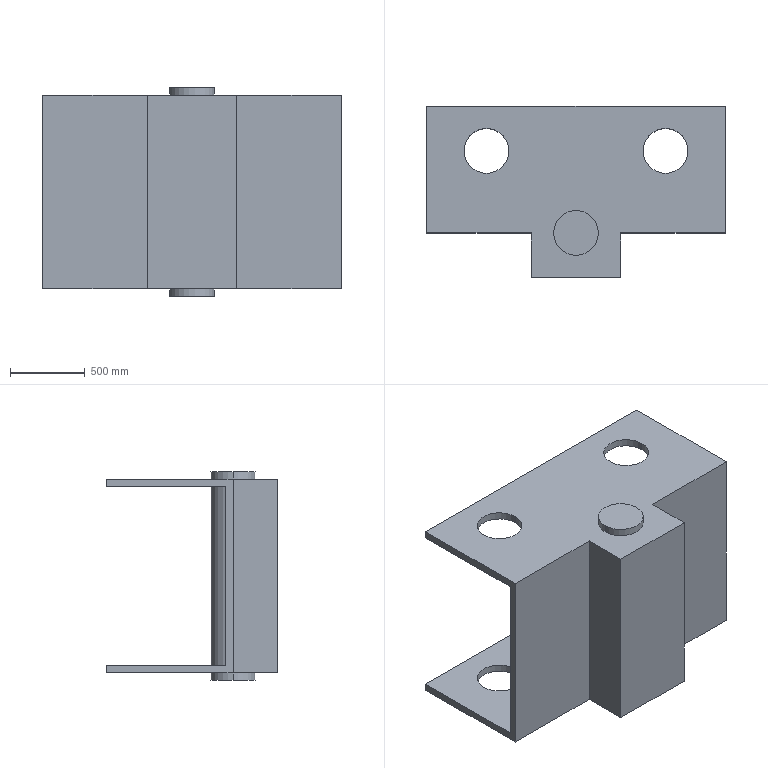Component | SolidWorks | RunningMechanism-4_Part12-2 | 1 solid | 34 faces | box 2000 x 1150 x 1400 mm | volume 421754418 mm3 | plane 20 | cylinder 14 | commonest cylinder face diameters 300 x14
build123d program:
from build123d import *

# Parameters (mm, degrees)
BOSS_EXTRUDE1_DEPTH = 650
SHELL1_T            = -50
SKETCH2_R           = 150
CUT_EXTRUDE1_DEPTH  = 1300
BOSS_EXTRUDE2_START = 50
SKETCH3_R           = 150
BOSS_EXTRUDE2_DEPTH = 1400


with BuildPart() as part:
    # Sketch1 → Boss-Extrude1 (new, symmetric)
    with BuildSketch(Plane(origin=(0, 0, 0), x_dir=(0, 0, -1), z_dir=(1, 0, 0))):
        Polygon((-300, 425), (-300, 725), (300, 725), (300, 425), (1000, 425), (1000, -425), (-1000, -425), (-1000, 425), align=None)
    extrude(amount=BOSS_EXTRUDE1_DEPTH, both=True)

    # Shell1
    shell1_openings = [part.faces().sort_by_distance(p)[0] for p in [
        (0, 0, 1000),
        (0, -425, 0),
        (0, 0, -1000),
    ]]
    offset(amount=SHELL1_T, openings=shell1_openings, kind=Kind.INTERSECTION)

    # Sketch2 → Cut-Extrude1 (cut)
    with BuildSketch(Plane(origin=(650, 0, 0), x_dir=(0, 0, -1), z_dir=(1, 0, 0))):
        with Locations((-600, -125)):
            Circle(SKETCH2_R)
    cut_extrude1 = extrude(amount=-CUT_EXTRUDE1_DEPTH, mode=Mode.SUBTRACT)

    # Mirror1: Cut-Extrude1 across plane
    add(cut_extrude1.mirror(Plane.XY), mode=Mode.SUBTRACT)

    # Sketch3 → Boss-Extrude2 (add)
    with BuildSketch(Plane(origin=(650, 0, 0), x_dir=(0, 0, -1), z_dir=(1, 0, 0)).offset(BOSS_EXTRUDE2_START)):
        with Locations((0, 425)):
            Circle(SKETCH3_R)
    extrude(amount=-BOSS_EXTRUDE2_DEPTH)


solid = part.part

# Placed as in the assembly
solid = solid.moved(Location((-4958.959, 55273.441, 24073.005), (180, 90, 0)))
STEP:
#1=COLOUR_RGB('',0.7922,0.8196,0.9333);
#2=FILL_AREA_STYLE_COLOUR('',#1);
#3=FILL_AREA_STYLE('',(#2));
#4=SURFACE_STYLE_FILL_AREA(#3);
#5=SURFACE_SIDE_STYLE('',(#4));
#6=SURFACE_STYLE_USAGE(.BOTH.,#5);
#7=PRESENTATION_STYLE_ASSIGNMENT((#6));
#8=CARTESIAN_POINT('',(-201.14,2159.387,973.347));
#9=VERTEX_POINT('',#8);
#10=CARTESIAN_POINT('',(-189.329,2159.387,973.347));
#11=VERTEX_POINT('',#10);
#12=CARTESIAN_POINT('',(-195.235,2159.387,973.347));
#13=DIRECTION('',(0.0000002,-0.,1.));
#14=DIRECTION('',(-1.,0.,0.0000002));
#15=AXIS2_PLACEMENT_3D('',#12,#13,#14);
#16=CIRCLE('',#15,5.906);
#17=EDGE_CURVE('',#9,#11,#16,.T.);
#18=ORIENTED_EDGE('',*,*,#17,.T.);
#19=CARTESIAN_POINT('',(-189.329,2159.387,975.315));
#20=VERTEX_POINT('',#19);
#21=CARTESIAN_POINT('',(-189.329,2159.387,920.197));
#22=DIRECTION('',(0.0000002,-0.,1.));
#23=VECTOR('',#22,39.37);
#24=LINE('',#21,#23);
#25=EDGE_CURVE('',#11,#20,#24,.T.);
#26=ORIENTED_EDGE('',*,*,#25,.T.);
#27=CARTESIAN_POINT('',(-201.14,2159.387,975.315));
#28=VERTEX_POINT('',#27);
#29=CARTESIAN_POINT('',(-195.235,2159.387,975.315));
#30=DIRECTION('',(0.0000002,-0.,1.));
#31=DIRECTION('',(-1.,0.,0.0000002));
#32=AXIS2_PLACEMENT_3D('',#29,#30,#31);
#33=CIRCLE('',#32,5.906);
#34=EDGE_CURVE('',#28,#20,#33,.T.);
#35=ORIENTED_EDGE('',*,*,#34,.F.);
#36=CARTESIAN_POINT('',(-201.14,2159.387,920.197));
#37=DIRECTION('',(0.0000002,-0.,1.));
#38=VECTOR('',#37,39.37);
#39=LINE('',#36,#38);
#40=EDGE_CURVE('',#9,#28,#39,.T.);
#41=ORIENTED_EDGE('',*,*,#40,.F.);
#42=EDGE_LOOP('',(#18,#26,#35,#41));
#43=FACE_OUTER_BOUND('',#42,.T.);
#44=CARTESIAN_POINT('',(-195.235,2159.387,920.197));
#45=DIRECTION('',(0.0000002,-0.,1.));
#46=DIRECTION('',(-1.,0.,0.0000002));
#47=AXIS2_PLACEMENT_3D('',#44,#45,#46);
#48=CYLINDRICAL_SURFACE('',#47,5.906);
#49=ADVANCED_FACE('',(#43),#48,.T.);
#50=CARTESIAN_POINT('',(-201.14,2159.387,920.197));
#51=VERTEX_POINT('',#50);
#52=CARTESIAN_POINT('',(-189.329,2159.387,920.197));
#53=VERTEX_POINT('',#52);
#54=CARTESIAN_POINT('',(-195.235,2159.387,920.197));
#55=DIRECTION('',(0.0000002,-0.,1.));
#56=DIRECTION('',(-1.,0.,0.0000002));
#57=AXIS2_PLACEMENT_3D('',#54,#55,#56);
#58=CIRCLE('',#57,5.906);
#59=EDGE_CURVE('',#51,#53,#58,.T.);
#60=ORIENTED_EDGE('',*,*,#59,.T.);
#61=CARTESIAN_POINT('',(-189.329,2159.387,922.166));
#62=VERTEX_POINT('',#61);
#63=CARTESIAN_POINT('',(-189.329,2159.387,920.197));
#64=DIRECTION('',(0.0000002,-0.,1.));
#65=VECTOR('',#64,39.37);
#66=LINE('',#63,#65);
#67=EDGE_CURVE('',#53,#62,#66,.T.);
#68=ORIENTED_EDGE('',*,*,#67,.T.);
#69=CARTESIAN_POINT('',(-201.14,2159.387,922.166));
#70=VERTEX_POINT('',#69);
#71=CARTESIAN_POINT('',(-195.235,2159.387,922.166));
#72=DIRECTION('',(0.0000002,-0.,1.));
#73=DIRECTION('',(-1.,0.,0.0000002));
#74=AXIS2_PLACEMENT_3D('',#71,#72,#73);
#75=CIRCLE('',#74,5.906);
#76=EDGE_CURVE('',#70,#62,#75,.T.);
#77=ORIENTED_EDGE('',*,*,#76,.F.);
#78=CARTESIAN_POINT('',(-201.14,2159.387,920.197));
#79=DIRECTION('',(0.0000002,-0.,1.));
#80=VECTOR('',#79,39.37);
#81=LINE('',#78,#80);
#82=EDGE_CURVE('',#51,#70,#81,.T.);
#83=ORIENTED_EDGE('',*,*,#82,.F.);
#84=EDGE_LOOP('',(#60,#68,#77,#83));
#85=FACE_OUTER_BOUND('',#84,.T.);
#86=CARTESIAN_POINT('',(-195.235,2159.387,920.197));
#87=DIRECTION('',(0.0000002,-0.,1.));
#88=DIRECTION('',(-1.,0.,0.0000002));
#89=AXIS2_PLACEMENT_3D('',#86,#87,#88);
#90=CYLINDRICAL_SURFACE('',#89,5.906);
#91=ADVANCED_FACE('',(#85),#90,.T.);
#92=CARTESIAN_POINT('',(-201.14,2159.387,924.134));
#93=VERTEX_POINT('',#92);
#94=CARTESIAN_POINT('',(-189.329,2159.387,924.134));
#95=VERTEX_POINT('',#94);
#96=CARTESIAN_POINT('',(-195.235,2159.387,924.134));
#97=DIRECTION('',(0.0000002,-0.,1.));
#98=DIRECTION('',(-1.,0.,0.0000002));
#99=AXIS2_PLACEMENT_3D('',#96,#97,#98);
#100=CIRCLE('',#99,5.906);
#101=EDGE_CURVE('',#93,#95,#100,.T.);
#102=ORIENTED_EDGE('',*,*,#101,.T.);
#103=CARTESIAN_POINT('',(-189.329,2159.387,971.378));
#104=VERTEX_POINT('',#103);
#105=CARTESIAN_POINT('',(-189.329,2159.387,920.197));
#106=DIRECTION('',(0.0000002,-0.,1.));
#107=VECTOR('',#106,39.37);
#108=LINE('',#105,#107);
#109=EDGE_CURVE('',#95,#104,#108,.T.);
#110=ORIENTED_EDGE('',*,*,#109,.T.);
#111=CARTESIAN_POINT('',(-201.14,2159.387,971.378));
#112=VERTEX_POINT('',#111);
#113=CARTESIAN_POINT('',(-195.235,2159.387,971.378));
#114=DIRECTION('',(0.0000002,-0.,1.));
#115=DIRECTION('',(-1.,0.,0.0000002));
#116=AXIS2_PLACEMENT_3D('',#113,#114,#115);
#117=CIRCLE('',#116,5.906);
#118=EDGE_CURVE('',#112,#104,#117,.T.);
#119=ORIENTED_EDGE('',*,*,#118,.F.);
#120=CARTESIAN_POINT('',(-201.14,2159.387,920.197));
#121=DIRECTION('',(0.0000002,-0.,1.));
#122=VECTOR('',#121,39.37);
#123=LINE('',#120,#122);
#124=EDGE_CURVE('',#93,#112,#123,.T.);
#125=ORIENTED_EDGE('',*,*,#124,.F.);
#126=EDGE_LOOP('',(#102,#110,#119,#125));
#127=FACE_OUTER_BOUND('',#126,.T.);
#128=CARTESIAN_POINT('',(-195.235,2159.387,920.197));
#129=DIRECTION('',(0.0000002,-0.,1.));
#130=DIRECTION('',(-1.,0.,0.0000002));
#131=AXIS2_PLACEMENT_3D('',#128,#129,#130);
#132=CYLINDRICAL_SURFACE('',#131,5.906);
#133=ADVANCED_FACE('',(#127),#132,.T.);
#134=CARTESIAN_POINT('',(-224.762,2181.041,971.378));
#135=VERTEX_POINT('',#134);
#136=CARTESIAN_POINT('',(-212.951,2181.041,971.378));
#137=VERTEX_POINT('',#136);
#138=CARTESIAN_POINT('',(-218.857,2181.041,971.378));
#139=DIRECTION('',(-0.0000002,0.,-1.));
#140=DIRECTION('',(-1.,0.,0.0000002));
#141=AXIS2_PLACEMENT_3D('',#138,#139,#140);
#142=CIRCLE('',#141,5.906);
#143=EDGE_CURVE('',#135,#137,#142,.T.);
#144=ORIENTED_EDGE('',*,*,#143,.T.);
#145=CARTESIAN_POINT('',(-212.951,2181.041,973.347));
#146=VERTEX_POINT('',#145);
#147=CARTESIAN_POINT('',(-212.951,2181.041,922.166));
#148=DIRECTION('',(0.0000002,-0.,1.));
#149=VECTOR('',#148,39.37);
#150=LINE('',#147,#149);
#151=EDGE_CURVE('',#137,#146,#150,.T.);
#152=ORIENTED_EDGE('',*,*,#151,.T.);
#153=CARTESIAN_POINT('',(-224.762,2181.041,973.347));
#154=VERTEX_POINT('',#153);
#155=CARTESIAN_POINT('',(-218.857,2181.041,973.347));
#156=DIRECTION('',(-0.0000002,0.,-1.));
#157=DIRECTION('',(1.,0.,-0.0000002));
#158=AXIS2_PLACEMENT_3D('',#155,#156,#157);
#159=CIRCLE('',#158,5.906);
#160=EDGE_CURVE('',#154,#146,#159,.T.);
#161=ORIENTED_EDGE('',*,*,#160,.F.);
#162=CARTESIAN_POINT('',(-224.762,2181.041,922.166));
#163=DIRECTION('',(0.0000002,-0.,1.));
#164=VECTOR('',#163,39.37);
#165=LINE('',#162,#164);
#166=EDGE_CURVE('',#135,#154,#165,.T.);
#167=ORIENTED_EDGE('',*,*,#166,.F.);
#168=EDGE_LOOP('',(#144,#152,#161,#167));
#169=FACE_OUTER_BOUND('',#168,.T.);
#170=CARTESIAN_POINT('',(-218.857,2181.041,922.166));
#171=DIRECTION('',(0.0000002,-0.,1.));
#172=DIRECTION('',(-1.,0.,0.0000002));
#173=AXIS2_PLACEMENT_3D('',#170,#171,#172);
#174=CYLINDRICAL_SURFACE('',#173,5.906);
#175=ADVANCED_FACE('',(#169),#174,.F.);
#176=CARTESIAN_POINT('',(-224.762,2181.041,922.166));
#177=VERTEX_POINT('',#176);
#178=CARTESIAN_POINT('',(-212.951,2181.041,922.166));
#179=VERTEX_POINT('',#178);
#180=CARTESIAN_POINT('',(-218.857,2181.041,922.166));
#181=DIRECTION('',(-0.0000002,0.,-1.));
#182=DIRECTION('',(1.,0.,-0.0000002));
#183=AXIS2_PLACEMENT_3D('',#180,#181,#182);
#184=CIRCLE('',#183,5.906);
#185=EDGE_CURVE('',#177,#179,#184,.T.);
#186=ORIENTED_EDGE('',*,*,#185,.T.);
#187=CARTESIAN_POINT('',(-212.951,2181.041,924.134));
#188=VERTEX_POINT('',#187);
#189=CARTESIAN_POINT('',(-212.951,2181.041,922.166));
#190=DIRECTION('',(0.0000002,-0.,1.));
#191=VECTOR('',#190,39.37);
#192=LINE('',#189,#191);
#193=EDGE_CURVE('',#179,#188,#192,.T.);
#194=ORIENTED_EDGE('',*,*,#193,.T.);
#195=CARTESIAN_POINT('',(-224.762,2181.041,924.134));
#196=VERTEX_POINT('',#195);
#197=CARTESIAN_POINT('',(-218.857,2181.041,924.134));
#198=DIRECTION('',(-0.0000002,0.,-1.));
#199=DIRECTION('',(-1.,0.,0.0000002));
#200=AXIS2_PLACEMENT_3D('',#197,#198,#199);
#201=CIRCLE('',#200,5.906);
#202=EDGE_CURVE('',#196,#188,#201,.T.);
#203=ORIENTED_EDGE('',*,*,#202,.F.);
#204=CARTESIAN_POINT('',(-224.762,2181.041,922.166));
#205=DIRECTION('',(0.0000002,-0.,1.));
#206=VECTOR('',#205,39.37);
#207=LINE('',#204,#206);
#208=EDGE_CURVE('',#177,#196,#207,.T.);
#209=ORIENTED_EDGE('',*,*,#208,.F.);
#210=EDGE_LOOP('',(#186,#194,#203,#209));
#211=FACE_OUTER_BOUND('',#210,.T.);
#212=CARTESIAN_POINT('',(-218.857,2181.041,922.166));
#213=DIRECTION('',(0.0000002,-0.,1.));
#214=DIRECTION('',(-1.,0.,0.0000002));
#215=AXIS2_PLACEMENT_3D('',#212,#213,#214);
#216=CYLINDRICAL_SURFACE('',#215,5.906);
#217=ADVANCED_FACE('',(#211),#216,.F.);
#218=CARTESIAN_POINT('',(-165.707,2181.041,971.378));
#219=VERTEX_POINT('',#218);
#220=CARTESIAN_POINT('',(-177.518,2181.041,971.378));
#221=VERTEX_POINT('',#220);
#222=CARTESIAN_POINT('',(-171.613,2181.041,971.378));
#223=DIRECTION('',(0.0000002,-0.,1.));
#224=DIRECTION('',(-1.,0.,0.0000002));
#225=AXIS2_PLACEMENT_3D('',#222,#223,#224);
#226=CIRCLE('',#225,5.906);
#227=EDGE_CURVE('',#219,#221,#226,.T.);
#228=ORIENTED_EDGE('',*,*,#227,.F.);
#229=CARTESIAN_POINT('',(-165.707,2181.041,973.347));
#230=VERTEX_POINT('',#229);
#231=CARTESIAN_POINT('',(-165.707,2181.041,922.166));
#232=DIRECTION('',(0.0000002,-0.,1.));
#233=VECTOR('',#232,39.37);
#234=LINE('',#231,#233);
#235=EDGE_CURVE('',#219,#230,#234,.T.);
#236=ORIENTED_EDGE('',*,*,#235,.T.);
#237=CARTESIAN_POINT('',(-177.518,2181.041,973.347));
#238=VERTEX_POINT('',#237);
#239=CARTESIAN_POINT('',(-171.613,2181.041,973.347));
#240=DIRECTION('',(0.0000002,-0.,1.));
#241=DIRECTION('',(-1.,0.,0.0000002));
#242=AXIS2_PLACEMENT_3D('',#239,#240,#241);
#243=CIRCLE('',#242,5.906);
#244=EDGE_CURVE('',#230,#238,#243,.T.);
#245=ORIENTED_EDGE('',*,*,#244,.T.);
#246=CARTESIAN_POINT('',(-177.518,2181.041,922.166));
#247=DIRECTION('',(0.0000002,-0.,1.));
#248=VECTOR('',#247,39.37);
#249=LINE('',#246,#248);
#250=EDGE_CURVE('',#221,#238,#249,.T.);
#251=ORIENTED_EDGE('',*,*,#250,.F.);
#252=EDGE_LOOP('',(#228,#236,#245,#251));
#253=FACE_OUTER_BOUND('',#252,.T.);
#254=CARTESIAN_POINT('',(-171.613,2181.041,922.166));
#255=DIRECTION('',(0.0000002,-0.,1.));
#256=DIRECTION('',(-1.,0.,0.0000002));
#257=AXIS2_PLACEMENT_3D('',#254,#255,#256);
#258=CYLINDRICAL_SURFACE('',#257,5.906);
#259=ADVANCED_FACE('',(#253),#258,.F.);
#260=CARTESIAN_POINT('',(-165.707,2181.041,922.166));
#261=VERTEX_POINT('',#260);
#262=CARTESIAN_POINT('',(-177.518,2181.041,922.166));
#263=VERTEX_POINT('',#262);
#264=CARTESIAN_POINT('',(-171.613,2181.041,922.166));
#265=DIRECTION('',(0.0000002,-0.,1.));
#266=DIRECTION('',(-1.,0.,0.0000002));
#267=AXIS2_PLACEMENT_3D('',#264,#265,#266);
#268=CIRCLE('',#267,5.906);
#269=EDGE_CURVE('',#261,#263,#268,.T.);
#270=ORIENTED_EDGE('',*,*,#269,.F.);
#271=CARTESIAN_POINT('',(-165.707,2181.041,924.134));
#272=VERTEX_POINT('',#271);
#273=CARTESIAN_POINT('',(-165.707,2181.041,922.166));
#274=DIRECTION('',(0.0000002,-0.,1.));
#275=VECTOR('',#274,39.37);
#276=LINE('',#273,#275);
#277=EDGE_CURVE('',#261,#272,#276,.T.);
#278=ORIENTED_EDGE('',*,*,#277,.T.);
#279=CARTESIAN_POINT('',(-177.518,2181.041,924.134));
#280=VERTEX_POINT('',#279);
#281=CARTESIAN_POINT('',(-171.613,2181.041,924.134));
#282=DIRECTION('',(0.0000002,-0.,1.));
#283=DIRECTION('',(-1.,0.,0.0000002));
#284=AXIS2_PLACEMENT_3D('',#281,#282,#283);
#285=CIRCLE('',#284,5.906);
#286=EDGE_CURVE('',#272,#280,#285,.T.);
#287=ORIENTED_EDGE('',*,*,#286,.T.);
#288=CARTESIAN_POINT('',(-177.518,2181.041,922.166));
#289=DIRECTION('',(0.0000002,-0.,1.));
#290=VECTOR('',#289,39.37);
#291=LINE('',#288,#290);
#292=EDGE_CURVE('',#263,#280,#291,.T.);
#293=ORIENTED_EDGE('',*,*,#292,.F.);
#294=EDGE_LOOP('',(#270,#278,#287,#293));
#295=FACE_OUTER_BOUND('',#294,.T.);
#296=CARTESIAN_POINT('',(-171.613,2181.041,922.166));
#297=DIRECTION('',(0.0000002,-0.,1.));
#298=DIRECTION('',(-1.,0.,0.0000002));
#299=AXIS2_PLACEMENT_3D('',#296,#297,#298);
#300=CYLINDRICAL_SURFACE('',#299,5.906);
#301=ADVANCED_FACE('',(#295),#300,.F.);
#302=CARTESIAN_POINT('',(-155.865,2161.356,924.134));
#303=VERTEX_POINT('',#302);
#304=CARTESIAN_POINT('',(-155.865,2192.852,924.134));
#305=VERTEX_POINT('',#304);
#306=CARTESIAN_POINT('',(-155.865,2192.852,924.134));
#307=DIRECTION('',(-0.,1.,0.));
#308=VECTOR('',#307,39.37);
#309=LINE('',#306,#308);
#310=EDGE_CURVE('',#303,#305,#309,.T.);
#311=ORIENTED_EDGE('',*,*,#310,.F.);
#312=CARTESIAN_POINT('',(-155.865,2161.356,971.378));
#313=VERTEX_POINT('',#312);
#314=CARTESIAN_POINT('',(-155.865,2161.356,973.347));
#315=DIRECTION('',(-0.0000002,0.,-1.));
#316=VECTOR('',#315,39.37);
#317=LINE('',#314,#316);
#318=EDGE_CURVE('',#313,#303,#317,.T.);
#319=ORIENTED_EDGE('',*,*,#318,.F.);
#320=CARTESIAN_POINT('',(-155.865,2192.852,971.378));
#321=VERTEX_POINT('',#320);
#322=CARTESIAN_POINT('',(-155.865,2192.852,971.378));
#323=DIRECTION('',(-0.,1.,0.));
#324=VECTOR('',#323,39.37);
#325=LINE('',#322,#324);
#326=EDGE_CURVE('',#313,#321,#325,.T.);
#327=ORIENTED_EDGE('',*,*,#326,.T.);
#328=CARTESIAN_POINT('',(-155.865,2192.852,973.347));
#329=VERTEX_POINT('',#328);
#330=CARTESIAN_POINT('',(-155.865,2192.852,973.347));
#331=DIRECTION('',(-0.0000002,0.,-1.));
#332=VECTOR('',#331,39.37);
#333=LINE('',#330,#332);
#334=EDGE_CURVE('',#329,#321,#333,.T.);
#335=ORIENTED_EDGE('',*,*,#334,.F.);
#336=CARTESIAN_POINT('',(-155.865,2159.387,973.347));
#337=VERTEX_POINT('',#336);
#338=CARTESIAN_POINT('',(-155.865,2192.852,973.347));
#339=DIRECTION('',(-0.,1.,0.));
#340=VECTOR('',#339,39.37);
#341=LINE('',#338,#340);
#342=EDGE_CURVE('',#337,#329,#341,.T.);
#343=ORIENTED_EDGE('',*,*,#342,.F.);
#344=CARTESIAN_POINT('',(-155.865,2159.387,922.166));
#345=VERTEX_POINT('',#344);
#346=CARTESIAN_POINT('',(-155.865,2159.387,973.347));
#347=DIRECTION('',(-0.0000002,0.,-1.));
#348=VECTOR('',#347,39.37);
#349=LINE('',#346,#348);
#350=EDGE_CURVE('',#337,#345,#349,.T.);
#351=ORIENTED_EDGE('',*,*,#350,.T.);
#352=CARTESIAN_POINT('',(-155.865,2192.852,922.166));
#353=VERTEX_POINT('',#352);
#354=CARTESIAN_POINT('',(-155.865,2192.852,922.166));
#355=DIRECTION('',(-0.,1.,0.));
#356=VECTOR('',#355,39.37);
#357=LINE('',#354,#356);
#358=EDGE_CURVE('',#345,#353,#357,.T.);
#359=ORIENTED_EDGE('',*,*,#358,.T.);
#360=CARTESIAN_POINT('',(-155.865,2192.852,973.347));
#361=DIRECTION('',(-0.0000002,0.,-1.));
#362=VECTOR('',#361,39.37);
#363=LINE('',#360,#362);
#364=EDGE_CURVE('',#305,#353,#363,.T.);
#365=ORIENTED_EDGE('',*,*,#364,.F.);
#366=EDGE_LOOP('',(#311,#319,#327,#335,#343,#351,#359,#365));
#367=FACE_OUTER_BOUND('',#366,.T.);
#368=CARTESIAN_POINT('',(-155.865,2192.852,973.347));
#369=DIRECTION('',(-1.,-0.,0.0000002));
#370=DIRECTION('',(-0.0000002,0.,-1.));
#371=AXIS2_PLACEMENT_3D('',#368,#369,#370);
#372=PLANE('',#371);
#373=ADVANCED_FACE('',(#367),#372,.F.);
#374=CARTESIAN_POINT('',(-234.605,2192.852,924.134));
#375=VERTEX_POINT('',#374);
#376=CARTESIAN_POINT('',(-155.865,2192.852,924.134));
#377=DIRECTION('',(-1.,-0.,0.0000002));
#378=VECTOR('',#377,39.37);
#379=LINE('',#376,#378);
#380=EDGE_CURVE('',#305,#375,#379,.T.);
#381=ORIENTED_EDGE('',*,*,#380,.F.);
#382=ORIENTED_EDGE('',*,*,#364,.T.);
#383=CARTESIAN_POINT('',(-234.605,2192.852,922.166));
#384=VERTEX_POINT('',#383);
#385=CARTESIAN_POINT('',(-155.865,2192.852,922.166));
#386=DIRECTION('',(-1.,-0.,0.0000002));
#387=VECTOR('',#386,39.37);
#388=LINE('',#385,#387);
#389=EDGE_CURVE('',#353,#384,#388,.T.);
#390=ORIENTED_EDGE('',*,*,#389,.T.);
#391=CARTESIAN_POINT('',(-234.605,2192.852,973.347));
#392=DIRECTION('',(-0.0000002,0.,-1.));
#393=VECTOR('',#392,39.37);
#394=LINE('',#391,#393);
#395=EDGE_CURVE('',#375,#384,#394,.T.);
#396=ORIENTED_EDGE('',*,*,#395,.F.);
#397=EDGE_LOOP('',(#381,#382,#390,#396));
#398=FACE_OUTER_BOUND('',#397,.T.);
#399=CARTESIAN_POINT('',(-155.865,2192.852,973.347));
#400=DIRECTION('',(0.,-1.,-0.));
#401=DIRECTION('',(1.,0.,-0.0000002));
#402=AXIS2_PLACEMENT_3D('',#399,#400,#401);
#403=PLANE('',#402);
#404=ADVANCED_FACE('',(#398),#403,.F.);
#405=CARTESIAN_POINT('',(-234.605,2161.356,924.134));
#406=VERTEX_POINT('',#405);
#407=CARTESIAN_POINT('',(-234.605,2192.852,924.134));
#408=DIRECTION('',(0.,-1.,-0.));
#409=VECTOR('',#408,39.37);
#410=LINE('',#407,#409);
#411=EDGE_CURVE('',#375,#406,#410,.T.);
#412=ORIENTED_EDGE('',*,*,#411,.F.);
#413=ORIENTED_EDGE('',*,*,#395,.T.);
#414=CARTESIAN_POINT('',(-234.605,2159.387,922.166));
#415=VERTEX_POINT('',#414);
#416=CARTESIAN_POINT('',(-234.605,2192.852,922.166));
#417=DIRECTION('',(0.,-1.,-0.));
#418=VECTOR('',#417,39.37);
#419=LINE('',#416,#418);
#420=EDGE_CURVE('',#384,#415,#419,.T.);
#421=ORIENTED_EDGE('',*,*,#420,.T.);
#422=CARTESIAN_POINT('',(-234.605,2159.387,973.347));
#423=VERTEX_POINT('',#422);
#424=CARTESIAN_POINT('',(-234.605,2159.387,973.347));
#425=DIRECTION('',(-0.0000002,0.,-1.));
#426=VECTOR('',#425,39.37);
#427=LINE('',#424,#426);
#428=EDGE_CURVE('',#423,#415,#427,.T.);
#429=ORIENTED_EDGE('',*,*,#428,.F.);
#430=CARTESIAN_POINT('',(-234.605,2192.852,973.347));
#431=VERTEX_POINT('',#430);
#432=CARTESIAN_POINT('',(-234.605,2192.852,973.347));
#433=DIRECTION('',(0.,-1.,-0.));
#434=VECTOR('',#433,39.37);
#435=LINE('',#432,#434);
#436=EDGE_CURVE('',#431,#423,#435,.T.);
#437=ORIENTED_EDGE('',*,*,#436,.F.);
#438=CARTESIAN_POINT('',(-234.605,2192.852,971.378));
#439=VERTEX_POINT('',#438);
#440=CARTESIAN_POINT('',(-234.605,2192.852,973.347));
#441=DIRECTION('',(-0.0000002,0.,-1.));
#442=VECTOR('',#441,39.37);
#443=LINE('',#440,#442);
#444=EDGE_CURVE('',#431,#439,#443,.T.);
#445=ORIENTED_EDGE('',*,*,#444,.T.);
#446=CARTESIAN_POINT('',(-234.605,2161.356,971.378));
#447=VERTEX_POINT('',#446);
#448=CARTESIAN_POINT('',(-234.605,2192.852,971.378));
#449=DIRECTION('',(0.,-1.,-0.));
#450=VECTOR('',#449,39.37);
#451=LINE('',#448,#450);
#452=EDGE_CURVE('',#439,#447,#451,.T.);
#453=ORIENTED_EDGE('',*,*,#452,.T.);
#454=CARTESIAN_POINT('',(-234.605,2161.356,973.347));
#455=DIRECTION('',(-0.0000002,0.,-1.));
#456=VECTOR('',#455,39.37);
#457=LINE('',#454,#456);
#458=EDGE_CURVE('',#447,#406,#457,.T.);
#459=ORIENTED_EDGE('',*,*,#458,.T.);
#460=EDGE_LOOP('',(#412,#413,#421,#429,#437,#445,#453,#459));
#461=FACE_OUTER_BOUND('',#460,.T.);
#462=CARTESIAN_POINT('',(-234.605,2192.852,973.347));
#463=DIRECTION('',(1.,0.,-0.0000002));
#464=DIRECTION('',(0.0000002,-0.,1.));
#465=AXIS2_PLACEMENT_3D('',#462,#463,#464);
#466=PLANE('',#465);
#467=ADVANCED_FACE('',(#461),#466,.F.);
#468=CARTESIAN_POINT('',(-207.046,2159.387,922.166));
#469=VERTEX_POINT('',#468);
#470=CARTESIAN_POINT('',(-207.046,2159.387,922.166));
#471=DIRECTION('',(1.,0.,-0.0000002));
#472=VECTOR('',#471,39.37);
#473=LINE('',#470,#472);
#474=EDGE_CURVE('',#415,#469,#473,.T.);
#475=ORIENTED_EDGE('',*,*,#474,.T.);
#476=CARTESIAN_POINT('',(-207.046,2159.387,973.347));
#477=VERTEX_POINT('',#476);
#478=CARTESIAN_POINT('',(-207.046,2159.387,973.347));
#479=DIRECTION('',(-0.0000002,0.,-1.));
#480=VECTOR('',#479,39.37);
#481=LINE('',#478,#480);
#482=EDGE_CURVE('',#477,#469,#481,.T.);
#483=ORIENTED_EDGE('',*,*,#482,.F.);
#484=CARTESIAN_POINT('',(-207.046,2159.387,973.347));
#485=DIRECTION('',(1.,0.,-0.0000002));
#486=VECTOR('',#485,39.37);
#487=LINE('',#484,#486);
#488=EDGE_CURVE('',#423,#477,#487,.T.);
#489=ORIENTED_EDGE('',*,*,#488,.F.);
#490=ORIENTED_EDGE('',*,*,#428,.T.);
#491=EDGE_LOOP('',(#475,#483,#489,#490));
#492=FACE_OUTER_BOUND('',#491,.T.);
#493=CARTESIAN_POINT('',(-207.046,2159.387,973.347));
#494=DIRECTION('',(-0.,1.,0.));
#495=DIRECTION('',(-1.,-0.,0.0000002));
#496=AXIS2_PLACEMENT_3D('',#493,#494,#495);
#497=PLANE('',#496);
#498=ADVANCED_FACE('',(#492),#497,.F.);
#499=CARTESIAN_POINT('',(-207.046,2147.576,922.166));
#500=VERTEX_POINT('',#499);
#501=CARTESIAN_POINT('',(-207.046,2147.576,922.166));
#502=DIRECTION('',(-0.,-1.,-0.));
#503=VECTOR('',#502,39.37);
#504=LINE('',#501,#503);
#505=EDGE_CURVE('',#469,#500,#504,.T.);
#506=ORIENTED_EDGE('',*,*,#505,.T.);
#507=CARTESIAN_POINT('',(-207.046,2147.576,973.347));
#508=VERTEX_POINT('',#507);
#509=CARTESIAN_POINT('',(-207.046,2147.576,973.347));
#510=DIRECTION('',(-0.0000002,0.,-1.));
#511=VECTOR('',#510,39.37);
#512=LINE('',#509,#511);
#513=EDGE_CURVE('',#508,#500,#512,.T.);
#514=ORIENTED_EDGE('',*,*,#513,.F.);
#515=CARTESIAN_POINT('',(-207.046,2147.576,973.347));
#516=DIRECTION('',(-0.,-1.,-0.));
#517=VECTOR('',#516,39.37);
#518=LINE('',#515,#517);
#519=EDGE_CURVE('',#477,#508,#518,.T.);
#520=ORIENTED_EDGE('',*,*,#519,.F.);
#521=ORIENTED_EDGE('',*,*,#482,.T.);
#522=EDGE_LOOP('',(#506,#514,#520,#521));
#523=FACE_OUTER_BOUND('',#522,.T.);
#524=CARTESIAN_POINT('',(-207.046,2147.576,973.347));
#525=DIRECTION('',(1.,-0.,-0.0000002));
#526=DIRECTION('',(0.,1.,0.));
#527=AXIS2_PLACEMENT_3D('',#524,#525,#526);
#528=PLANE('',#527);
#529=ADVANCED_FACE('',(#523),#528,.F.);
#530=CARTESIAN_POINT('',(-183.424,2147.576,922.166));
#531=VERTEX_POINT('',#530);
#532=CARTESIAN_POINT('',(-183.424,2147.576,922.166));
#533=DIRECTION('',(1.,0.,-0.0000002));
#534=VECTOR('',#533,39.37);
#535=LINE('',#532,#534);
#536=EDGE_CURVE('',#500,#531,#535,.T.);
#537=ORIENTED_EDGE('',*,*,#536,.T.);
#538=CARTESIAN_POINT('',(-183.424,2147.576,973.347));
#539=VERTEX_POINT('',#538);
#540=CARTESIAN_POINT('',(-183.424,2147.576,973.347));
#541=DIRECTION('',(-0.0000002,0.,-1.));
#542=VECTOR('',#541,39.37);
#543=LINE('',#540,#542);
#544=EDGE_CURVE('',#539,#531,#543,.T.);
#545=ORIENTED_EDGE('',*,*,#544,.F.);
#546=CARTESIAN_POINT('',(-183.424,2147.576,973.347));
#547=DIRECTION('',(1.,0.,-0.0000002));
#548=VECTOR('',#547,39.37);
#549=LINE('',#546,#548);
#550=EDGE_CURVE('',#508,#539,#549,.T.);
#551=ORIENTED_EDGE('',*,*,#550,.F.);
#552=ORIENTED_EDGE('',*,*,#513,.T.);
#553=EDGE_LOOP('',(#537,#545,#551,#552));
#554=FACE_OUTER_BOUND('',#553,.T.);
#555=CARTESIAN_POINT('',(-183.424,2147.576,973.347));
#556=DIRECTION('',(-0.,1.,0.));
#557=DIRECTION('',(-1.,-0.,0.0000002));
#558=AXIS2_PLACEMENT_3D('',#555,#556,#557);
#559=PLANE('',#558);
#560=ADVANCED_FACE('',(#554),#559,.F.);
#561=CARTESIAN_POINT('',(-183.424,2159.387,922.166));
#562=VERTEX_POINT('',#561);
#563=CARTESIAN_POINT('',(-183.424,2159.387,922.166));
#564=DIRECTION('',(-0.,1.,0.));
#565=VECTOR('',#564,39.37);
#566=LINE('',#563,#565);
#567=EDGE_CURVE('',#531,#562,#566,.T.);
#568=ORIENTED_EDGE('',*,*,#567,.T.);
#569=CARTESIAN_POINT('',(-183.424,2159.387,973.347));
#570=VERTEX_POINT('',#569);
#571=CARTESIAN_POINT('',(-183.424,2159.387,973.347));
#572=DIRECTION('',(-0.0000002,0.,-1.));
#573=VECTOR('',#572,39.37);
#574=LINE('',#571,#573);
#575=EDGE_CURVE('',#570,#562,#574,.T.);
#576=ORIENTED_EDGE('',*,*,#575,.F.);
#577=CARTESIAN_POINT('',(-183.424,2159.387,973.347));
#578=DIRECTION('',(-0.,1.,0.));
#579=VECTOR('',#578,39.37);
#580=LINE('',#577,#579);
#581=EDGE_CURVE('',#539,#570,#580,.T.);
#582=ORIENTED_EDGE('',*,*,#581,.F.);
#583=ORIENTED_EDGE('',*,*,#544,.T.);
#584=EDGE_LOOP('',(#568,#576,#582,#583));
#585=FACE_OUTER_BOUND('',#584,.T.);
#586=CARTESIAN_POINT('',(-183.424,2159.387,973.347));
#587=DIRECTION('',(-1.,-0.,0.0000002));
#588=DIRECTION('',(0.,-1.,-0.));
#589=AXIS2_PLACEMENT_3D('',#586,#587,#588);
#590=PLANE('',#589);
#591=ADVANCED_FACE('',(#585),#590,.F.);
#592=CARTESIAN_POINT('',(-155.865,2159.387,922.166));
#593=DIRECTION('',(1.,0.,-0.0000002));
#594=VECTOR('',#593,39.37);
#595=LINE('',#592,#594);
#596=EDGE_CURVE('',#562,#345,#595,.T.);
#597=ORIENTED_EDGE('',*,*,#596,.T.);
#598=ORIENTED_EDGE('',*,*,#350,.F.);
#599=CARTESIAN_POINT('',(-155.865,2159.387,973.347));
#600=DIRECTION('',(1.,0.,-0.0000002));
#601=VECTOR('',#600,39.37);
#602=LINE('',#599,#601);
#603=EDGE_CURVE('',#570,#337,#602,.T.);
#604=ORIENTED_EDGE('',*,*,#603,.F.);
#605=ORIENTED_EDGE('',*,*,#575,.T.);
#606=EDGE_LOOP('',(#597,#598,#604,#605));
#607=FACE_OUTER_BOUND('',#606,.T.);
#608=CARTESIAN_POINT('',(-155.865,2159.387,973.347));
#609=DIRECTION('',(-0.,1.,0.));
#610=DIRECTION('',(-1.,-0.,0.0000002));
#611=AXIS2_PLACEMENT_3D('',#608,#609,#610);
#612=PLANE('',#611);
#613=ADVANCED_FACE('',(#607),#612,.F.);
#614=ORIENTED_EDGE('',*,*,#334,.T.);
#615=CARTESIAN_POINT('',(-155.865,2192.852,971.378));
#616=DIRECTION('',(-1.,-0.,0.0000002));
#617=VECTOR('',#616,39.37);
#618=LINE('',#615,#617);
#619=EDGE_CURVE('',#321,#439,#618,.T.);
#620=ORIENTED_EDGE('',*,*,#619,.T.);
#621=ORIENTED_EDGE('',*,*,#444,.F.);
#622=CARTESIAN_POINT('',(-155.865,2192.852,973.347));
#623=DIRECTION('',(-1.,-0.,0.0000002));
#624=VECTOR('',#623,39.37);
#625=LINE('',#622,#624);
#626=EDGE_CURVE('',#329,#431,#625,.T.);
#627=ORIENTED_EDGE('',*,*,#626,.F.);
#628=EDGE_LOOP('',(#614,#620,#621,#627));
#629=FACE_OUTER_BOUND('',#628,.T.);
#630=CARTESIAN_POINT('',(-155.865,2192.852,973.347));
#631=DIRECTION('',(0.,-1.,-0.));
#632=DIRECTION('',(1.,0.,-0.0000002));
#633=AXIS2_PLACEMENT_3D('',#630,#631,#632);
#634=PLANE('',#633);
#635=ADVANCED_FACE('',(#629),#634,.F.);
#636=ORIENTED_EDGE('',*,*,#17,.F.);
#637=CARTESIAN_POINT('',(-195.235,2159.387,973.347));
#638=DIRECTION('',(0.0000002,-0.,1.));
#639=DIRECTION('',(-1.,0.,0.0000002));
#640=AXIS2_PLACEMENT_3D('',#637,#638,#639);
#641=CIRCLE('',#640,5.906);
#642=EDGE_CURVE('',#11,#9,#641,.T.);
#643=ORIENTED_EDGE('',*,*,#642,.F.);
#644=EDGE_LOOP('',(#636,#643));
#645=FACE_BOUND('',#644,.T.);
#646=ORIENTED_EDGE('',*,*,#160,.T.);
#647=CARTESIAN_POINT('',(-218.857,2181.041,973.347));
#648=DIRECTION('',(-0.0000002,0.,-1.));
#649=DIRECTION('',(1.,0.,-0.0000002));
#650=AXIS2_PLACEMENT_3D('',#647,#648,#649);
#651=CIRCLE('',#650,5.906);
#652=EDGE_CURVE('',#146,#154,#651,.T.);
#653=ORIENTED_EDGE('',*,*,#652,.T.);
#654=EDGE_LOOP('',(#646,#653));
#655=FACE_BOUND('',#654,.T.);
#656=CARTESIAN_POINT('',(-171.613,2181.041,973.347));
#657=DIRECTION('',(0.0000002,-0.,1.));
#658=DIRECTION('',(-1.,0.,0.0000002));
#659=AXIS2_PLACEMENT_3D('',#656,#657,#658);
#660=CIRCLE('',#659,5.906);
#661=EDGE_CURVE('',#238,#230,#660,.T.);
#662=ORIENTED_EDGE('',*,*,#661,.F.);
#663=ORIENTED_EDGE('',*,*,#244,.F.);
#664=EDGE_LOOP('',(#662,#663));
#665=FACE_BOUND('',#664,.T.);
#666=ORIENTED_EDGE('',*,*,#488,.T.);
#667=ORIENTED_EDGE('',*,*,#519,.T.);
#668=ORIENTED_EDGE('',*,*,#550,.T.);
#669=ORIENTED_EDGE('',*,*,#581,.T.);
#670=ORIENTED_EDGE('',*,*,#603,.T.);
#671=ORIENTED_EDGE('',*,*,#342,.T.);
#672=ORIENTED_EDGE('',*,*,#626,.T.);
#673=ORIENTED_EDGE('',*,*,#436,.T.);
#674=EDGE_LOOP('',(#666,#667,#668,#669,#670,#671,#672,#673));
#675=FACE_OUTER_BOUND('',#674,.T.);
#676=CARTESIAN_POINT('',(-195.235,2176.12,973.347));
#677=DIRECTION('',(0.0000002,-0.,1.));
#678=DIRECTION('',(-1.,-0.,0.0000002));
#679=AXIS2_PLACEMENT_3D('',#676,#677,#678);
#680=PLANE('',#679);
#681=ADVANCED_FACE('',(#645,#655,#665,#675),#680,.T.);
#682=ORIENTED_EDGE('',*,*,#76,.T.);
#683=CARTESIAN_POINT('',(-195.235,2159.387,922.166));
#684=DIRECTION('',(0.0000002,-0.,1.));
#685=DIRECTION('',(-1.,0.,0.0000002));
#686=AXIS2_PLACEMENT_3D('',#683,#684,#685);
#687=CIRCLE('',#686,5.906);
#688=EDGE_CURVE('',#62,#70,#687,.T.);
#689=ORIENTED_EDGE('',*,*,#688,.T.);
#690=EDGE_LOOP('',(#682,#689));
#691=FACE_BOUND('',#690,.T.);
#692=ORIENTED_EDGE('',*,*,#185,.F.);
#693=CARTESIAN_POINT('',(-218.857,2181.041,922.166));
#694=DIRECTION('',(-0.0000002,0.,-1.));
#695=DIRECTION('',(1.,0.,-0.0000002));
#696=AXIS2_PLACEMENT_3D('',#693,#694,#695);
#697=CIRCLE('',#696,5.906);
#698=EDGE_CURVE('',#179,#177,#697,.T.);
#699=ORIENTED_EDGE('',*,*,#698,.F.);
#700=EDGE_LOOP('',(#692,#699));
#701=FACE_BOUND('',#700,.T.);
#702=CARTESIAN_POINT('',(-171.613,2181.041,922.166));
#703=DIRECTION('',(0.0000002,-0.,1.));
#704=DIRECTION('',(-1.,0.,0.0000002));
#705=AXIS2_PLACEMENT_3D('',#702,#703,#704);
#706=CIRCLE('',#705,5.906);
#707=EDGE_CURVE('',#263,#261,#706,.T.);
#708=ORIENTED_EDGE('',*,*,#707,.T.);
#709=ORIENTED_EDGE('',*,*,#269,.T.);
#710=EDGE_LOOP('',(#708,#709));
#711=FACE_BOUND('',#710,.T.);
#712=ORIENTED_EDGE('',*,*,#474,.F.);
#713=ORIENTED_EDGE('',*,*,#420,.F.);
#714=ORIENTED_EDGE('',*,*,#389,.F.);
#715=ORIENTED_EDGE('',*,*,#358,.F.);
#716=ORIENTED_EDGE('',*,*,#596,.F.);
#717=ORIENTED_EDGE('',*,*,#567,.F.);
#718=ORIENTED_EDGE('',*,*,#536,.F.);
#719=ORIENTED_EDGE('',*,*,#505,.F.);
#720=EDGE_LOOP('',(#712,#713,#714,#715,#716,#717,#718,#719));
#721=FACE_OUTER_BOUND('',#720,.T.);
#722=CARTESIAN_POINT('',(-195.235,2176.12,922.166));
#723=DIRECTION('',(0.0000002,-0.,1.));
#724=DIRECTION('',(-1.,-0.,0.0000002));
#725=AXIS2_PLACEMENT_3D('',#722,#723,#724);
#726=PLANE('',#725);
#727=ADVANCED_FACE('',(#691,#701,#711,#721),#726,.F.);
#728=CARTESIAN_POINT('',(-205.077,2161.356,924.134));
#729=VERTEX_POINT('',#728);
#730=CARTESIAN_POINT('',(-207.046,2161.356,924.134));
#731=DIRECTION('',(1.,0.,-0.0000002));
#732=VECTOR('',#731,39.37);
#733=LINE('',#730,#732);
#734=EDGE_CURVE('',#406,#729,#733,.T.);
#735=ORIENTED_EDGE('',*,*,#734,.F.);
#736=ORIENTED_EDGE('',*,*,#458,.F.);
#737=CARTESIAN_POINT('',(-205.077,2161.356,971.378));
#738=VERTEX_POINT('',#737);
#739=CARTESIAN_POINT('',(-207.046,2161.356,971.378));
#740=DIRECTION('',(1.,0.,-0.0000002));
#741=VECTOR('',#740,39.37);
#742=LINE('',#739,#741);
#743=EDGE_CURVE('',#447,#738,#742,.T.);
#744=ORIENTED_EDGE('',*,*,#743,.T.);
#745=CARTESIAN_POINT('',(-205.077,2161.356,973.347));
#746=DIRECTION('',(-0.0000002,0.,-1.));
#747=VECTOR('',#746,39.37);
#748=LINE('',#745,#747);
#749=EDGE_CURVE('',#738,#729,#748,.T.);
#750=ORIENTED_EDGE('',*,*,#749,.T.);
#751=EDGE_LOOP('',(#735,#736,#744,#750));
#752=FACE_OUTER_BOUND('',#751,.T.);
#753=CARTESIAN_POINT('',(-207.046,2161.356,973.347));
#754=DIRECTION('',(-0.,1.,0.));
#755=DIRECTION('',(-1.,-0.,0.0000002));
#756=AXIS2_PLACEMENT_3D('',#753,#754,#755);
#757=PLANE('',#756);
#758=ADVANCED_FACE('',(#752),#757,.T.);
#759=CARTESIAN_POINT('',(-205.077,2149.545,924.134));
#760=VERTEX_POINT('',#759);
#761=CARTESIAN_POINT('',(-205.077,2147.576,924.134));
#762=DIRECTION('',(-0.,-1.,-0.));
#763=VECTOR('',#762,39.37);
#764=LINE('',#761,#763);
#765=EDGE_CURVE('',#729,#760,#764,.T.);
#766=ORIENTED_EDGE('',*,*,#765,.F.);
#767=ORIENTED_EDGE('',*,*,#749,.F.);
#768=CARTESIAN_POINT('',(-205.077,2149.545,971.378));
#769=VERTEX_POINT('',#768);
#770=CARTESIAN_POINT('',(-205.077,2147.576,971.378));
#771=DIRECTION('',(-0.,-1.,-0.));
#772=VECTOR('',#771,39.37);
#773=LINE('',#770,#772);
#774=EDGE_CURVE('',#738,#769,#773,.T.);
#775=ORIENTED_EDGE('',*,*,#774,.T.);
#776=CARTESIAN_POINT('',(-205.077,2149.545,973.347));
#777=DIRECTION('',(-0.0000002,0.,-1.));
#778=VECTOR('',#777,39.37);
#779=LINE('',#776,#778);
#780=EDGE_CURVE('',#769,#760,#779,.T.);
#781=ORIENTED_EDGE('',*,*,#780,.T.);
#782=EDGE_LOOP('',(#766,#767,#775,#781));
#783=FACE_OUTER_BOUND('',#782,.T.);
#784=CARTESIAN_POINT('',(-205.077,2147.576,973.347));
#785=DIRECTION('',(1.,-0.,-0.0000002));
#786=DIRECTION('',(0.,1.,0.));
#787=AXIS2_PLACEMENT_3D('',#784,#785,#786);
#788=PLANE('',#787);
#789=ADVANCED_FACE('',(#783),#788,.T.);
#790=CARTESIAN_POINT('',(-185.392,2149.545,924.134));
#791=VERTEX_POINT('',#790);
#792=CARTESIAN_POINT('',(-183.424,2149.545,924.134));
#793=DIRECTION('',(1.,0.,-0.0000002));
#794=VECTOR('',#793,39.37);
#795=LINE('',#792,#794);
#796=EDGE_CURVE('',#760,#791,#795,.T.);
#797=ORIENTED_EDGE('',*,*,#796,.F.);
#798=ORIENTED_EDGE('',*,*,#780,.F.);
#799=CARTESIAN_POINT('',(-185.392,2149.545,971.378));
#800=VERTEX_POINT('',#799);
#801=CARTESIAN_POINT('',(-183.424,2149.545,971.378));
#802=DIRECTION('',(1.,0.,-0.0000002));
#803=VECTOR('',#802,39.37);
#804=LINE('',#801,#803);
#805=EDGE_CURVE('',#769,#800,#804,.T.);
#806=ORIENTED_EDGE('',*,*,#805,.T.);
#807=CARTESIAN_POINT('',(-185.392,2149.545,973.347));
#808=DIRECTION('',(-0.0000002,0.,-1.));
#809=VECTOR('',#808,39.37);
#810=LINE('',#807,#809);
#811=EDGE_CURVE('',#800,#791,#810,.T.);
#812=ORIENTED_EDGE('',*,*,#811,.T.);
#813=EDGE_LOOP('',(#797,#798,#806,#812));
#814=FACE_OUTER_BOUND('',#813,.T.);
#815=CARTESIAN_POINT('',(-183.424,2149.545,973.347));
#816=DIRECTION('',(-0.,1.,0.));
#817=DIRECTION('',(-1.,-0.,0.0000002));
#818=AXIS2_PLACEMENT_3D('',#815,#816,#817);
#819=PLANE('',#818);
#820=ADVANCED_FACE('',(#814),#819,.T.);
#821=CARTESIAN_POINT('',(-185.392,2161.356,924.134));
#822=VERTEX_POINT('',#821);
#823=CARTESIAN_POINT('',(-185.392,2159.387,924.134));
#824=DIRECTION('',(-0.,1.,0.));
#825=VECTOR('',#824,39.37);
#826=LINE('',#823,#825);
#827=EDGE_CURVE('',#791,#822,#826,.T.);
#828=ORIENTED_EDGE('',*,*,#827,.F.);
#829=ORIENTED_EDGE('',*,*,#811,.F.);
#830=CARTESIAN_POINT('',(-185.392,2161.356,971.378));
#831=VERTEX_POINT('',#830);
#832=CARTESIAN_POINT('',(-185.392,2159.387,971.378));
#833=DIRECTION('',(-0.,1.,0.));
#834=VECTOR('',#833,39.37);
#835=LINE('',#832,#834);
#836=EDGE_CURVE('',#800,#831,#835,.T.);
#837=ORIENTED_EDGE('',*,*,#836,.T.);
#838=CARTESIAN_POINT('',(-185.392,2161.356,973.347));
#839=DIRECTION('',(-0.0000002,0.,-1.));
#840=VECTOR('',#839,39.37);
#841=LINE('',#838,#840);
#842=EDGE_CURVE('',#831,#822,#841,.T.);
#843=ORIENTED_EDGE('',*,*,#842,.T.);
#844=EDGE_LOOP('',(#828,#829,#837,#843));
#845=FACE_OUTER_BOUND('',#844,.T.);
#846=CARTESIAN_POINT('',(-185.392,2159.387,973.347));
#847=DIRECTION('',(-1.,-0.,0.0000002));
#848=DIRECTION('',(0.,-1.,-0.));
#849=AXIS2_PLACEMENT_3D('',#846,#847,#848);
#850=PLANE('',#849);
#851=ADVANCED_FACE('',(#845),#850,.T.);
#852=CARTESIAN_POINT('',(-155.865,2161.356,924.134));
#853=DIRECTION('',(1.,0.,-0.0000002));
#854=VECTOR('',#853,39.37);
#855=LINE('',#852,#854);
#856=EDGE_CURVE('',#822,#303,#855,.T.);
#857=ORIENTED_EDGE('',*,*,#856,.F.);
#858=ORIENTED_EDGE('',*,*,#842,.F.);
#859=CARTESIAN_POINT('',(-155.865,2161.356,971.378));
#860=DIRECTION('',(1.,0.,-0.0000002));
#861=VECTOR('',#860,39.37);
#862=LINE('',#859,#861);
#863=EDGE_CURVE('',#831,#313,#862,.T.);
#864=ORIENTED_EDGE('',*,*,#863,.T.);
#865=ORIENTED_EDGE('',*,*,#318,.T.);
#866=EDGE_LOOP('',(#857,#858,#864,#865));
#867=FACE_OUTER_BOUND('',#866,.T.);
#868=CARTESIAN_POINT('',(-155.865,2161.356,973.347));
#869=DIRECTION('',(-0.,1.,0.));
#870=DIRECTION('',(-1.,-0.,0.0000002));
#871=AXIS2_PLACEMENT_3D('',#868,#869,#870);
#872=PLANE('',#871);
#873=ADVANCED_FACE('',(#867),#872,.T.);
#874=ORIENTED_EDGE('',*,*,#118,.T.);
#875=CARTESIAN_POINT('',(-195.235,2159.387,971.378));
#876=DIRECTION('',(0.0000002,-0.,1.));
#877=DIRECTION('',(-1.,0.,0.0000002));
#878=AXIS2_PLACEMENT_3D('',#875,#876,#877);
#879=CIRCLE('',#878,5.906);
#880=EDGE_CURVE('',#104,#112,#879,.T.);
#881=ORIENTED_EDGE('',*,*,#880,.T.);
#882=EDGE_LOOP('',(#874,#881));
#883=FACE_BOUND('',#882,.T.);
#884=ORIENTED_EDGE('',*,*,#143,.F.);
#885=CARTESIAN_POINT('',(-218.857,2181.041,971.378));
#886=DIRECTION('',(-0.0000002,0.,-1.));
#887=DIRECTION('',(-1.,0.,0.0000002));
#888=AXIS2_PLACEMENT_3D('',#885,#886,#887);
#889=CIRCLE('',#888,5.906);
#890=EDGE_CURVE('',#137,#135,#889,.T.);
#891=ORIENTED_EDGE('',*,*,#890,.F.);
#892=EDGE_LOOP('',(#884,#891));
#893=FACE_BOUND('',#892,.T.);
#894=CARTESIAN_POINT('',(-171.613,2181.041,971.378));
#895=DIRECTION('',(0.0000002,-0.,1.));
#896=DIRECTION('',(-1.,0.,0.0000002));
#897=AXIS2_PLACEMENT_3D('',#894,#895,#896);
#898=CIRCLE('',#897,5.906);
#899=EDGE_CURVE('',#221,#219,#898,.T.);
#900=ORIENTED_EDGE('',*,*,#899,.T.);
#901=ORIENTED_EDGE('',*,*,#227,.T.);
#902=EDGE_LOOP('',(#900,#901));
#903=FACE_BOUND('',#902,.T.);
#904=ORIENTED_EDGE('',*,*,#743,.F.);
#905=ORIENTED_EDGE('',*,*,#452,.F.);
#906=ORIENTED_EDGE('',*,*,#619,.F.);
#907=ORIENTED_EDGE('',*,*,#326,.F.);
#908=ORIENTED_EDGE('',*,*,#863,.F.);
#909=ORIENTED_EDGE('',*,*,#836,.F.);
#910=ORIENTED_EDGE('',*,*,#805,.F.);
#911=ORIENTED_EDGE('',*,*,#774,.F.);
#912=EDGE_LOOP('',(#904,#905,#906,#907,#908,#909,#910,#911));
#913=FACE_OUTER_BOUND('',#912,.T.);
#914=CARTESIAN_POINT('',(-195.235,2176.12,971.378));
#915=DIRECTION('',(0.0000002,-0.,1.));
#916=DIRECTION('',(-1.,-0.,0.0000002));
#917=AXIS2_PLACEMENT_3D('',#914,#915,#916);
#918=PLANE('',#917);
#919=ADVANCED_FACE('',(#883,#893,#903,#913),#918,.F.);
#920=ORIENTED_EDGE('',*,*,#101,.F.);
#921=CARTESIAN_POINT('',(-195.235,2159.387,924.134));
#922=DIRECTION('',(0.0000002,-0.,1.));
#923=DIRECTION('',(-1.,0.,0.0000002));
#924=AXIS2_PLACEMENT_3D('',#921,#922,#923);
#925=CIRCLE('',#924,5.906);
#926=EDGE_CURVE('',#95,#93,#925,.T.);
#927=ORIENTED_EDGE('',*,*,#926,.F.);
#928=EDGE_LOOP('',(#920,#927));
#929=FACE_BOUND('',#928,.T.);
#930=ORIENTED_EDGE('',*,*,#202,.T.);
#931=CARTESIAN_POINT('',(-218.857,2181.041,924.134));
#932=DIRECTION('',(-0.0000002,0.,-1.));
#933=DIRECTION('',(-1.,0.,0.0000002));
#934=AXIS2_PLACEMENT_3D('',#931,#932,#933);
#935=CIRCLE('',#934,5.906);
#936=EDGE_CURVE('',#188,#196,#935,.T.);
#937=ORIENTED_EDGE('',*,*,#936,.T.);
#938=EDGE_LOOP('',(#930,#937));
#939=FACE_BOUND('',#938,.T.);
#940=CARTESIAN_POINT('',(-171.613,2181.041,924.134));
#941=DIRECTION('',(0.0000002,-0.,1.));
#942=DIRECTION('',(-1.,0.,0.0000002));
#943=AXIS2_PLACEMENT_3D('',#940,#941,#942);
#944=CIRCLE('',#943,5.906);
#945=EDGE_CURVE('',#280,#272,#944,.T.);
#946=ORIENTED_EDGE('',*,*,#945,.F.);
#947=ORIENTED_EDGE('',*,*,#286,.F.);
#948=EDGE_LOOP('',(#946,#947));
#949=FACE_BOUND('',#948,.T.);
#950=ORIENTED_EDGE('',*,*,#734,.T.);
#951=ORIENTED_EDGE('',*,*,#765,.T.);
#952=ORIENTED_EDGE('',*,*,#796,.T.);
#953=ORIENTED_EDGE('',*,*,#827,.T.);
#954=ORIENTED_EDGE('',*,*,#856,.T.);
#955=ORIENTED_EDGE('',*,*,#310,.T.);
#956=ORIENTED_EDGE('',*,*,#380,.T.);
#957=ORIENTED_EDGE('',*,*,#411,.T.);
#958=EDGE_LOOP('',(#950,#951,#952,#953,#954,#955,#956,#957));
#959=FACE_OUTER_BOUND('',#958,.T.);
#960=CARTESIAN_POINT('',(-195.235,2176.12,924.134));
#961=DIRECTION('',(0.0000002,-0.,1.));
#962=DIRECTION('',(-1.,-0.,0.0000002));
#963=AXIS2_PLACEMENT_3D('',#960,#961,#962);
#964=PLANE('',#963);
#965=ADVANCED_FACE('',(#929,#939,#949,#959),#964,.T.);
#966=ORIENTED_EDGE('',*,*,#277,.F.);
#967=ORIENTED_EDGE('',*,*,#707,.F.);
#968=ORIENTED_EDGE('',*,*,#292,.T.);
#969=ORIENTED_EDGE('',*,*,#945,.T.);
#970=EDGE_LOOP('',(#966,#967,#968,#969));
#971=FACE_OUTER_BOUND('',#970,.T.);
#972=CARTESIAN_POINT('',(-171.613,2181.041,922.166));
#973=DIRECTION('',(0.0000002,-0.,1.));
#974=DIRECTION('',(-1.,0.,0.0000002));
#975=AXIS2_PLACEMENT_3D('',#972,#973,#974);
#976=CYLINDRICAL_SURFACE('',#975,5.906);
#977=ADVANCED_FACE('',(#971),#976,.F.);
#978=ORIENTED_EDGE('',*,*,#235,.F.);
#979=ORIENTED_EDGE('',*,*,#899,.F.);
#980=ORIENTED_EDGE('',*,*,#250,.T.);
#981=ORIENTED_EDGE('',*,*,#661,.T.);
#982=EDGE_LOOP('',(#978,#979,#980,#981));
#983=FACE_OUTER_BOUND('',#982,.T.);
#984=CARTESIAN_POINT('',(-171.613,2181.041,922.166));
#985=DIRECTION('',(0.0000002,-0.,1.));
#986=DIRECTION('',(-1.,0.,0.0000002));
#987=AXIS2_PLACEMENT_3D('',#984,#985,#986);
#988=CYLINDRICAL_SURFACE('',#987,5.906);
#989=ADVANCED_FACE('',(#983),#988,.F.);
#990=ORIENTED_EDGE('',*,*,#193,.F.);
#991=ORIENTED_EDGE('',*,*,#698,.T.);
#992=ORIENTED_EDGE('',*,*,#208,.T.);
#993=ORIENTED_EDGE('',*,*,#936,.F.);
#994=EDGE_LOOP('',(#990,#991,#992,#993));
#995=FACE_OUTER_BOUND('',#994,.T.);
#996=CARTESIAN_POINT('',(-218.857,2181.041,922.166));
#997=DIRECTION('',(0.0000002,-0.,1.));
#998=DIRECTION('',(-1.,0.,0.0000002));
#999=AXIS2_PLACEMENT_3D('',#996,#997,#998);
#1000=CYLINDRICAL_SURFACE('',#999,5.906);
#1001=ADVANCED_FACE('',(#995),#1000,.F.);
#1002=ORIENTED_EDGE('',*,*,#151,.F.);
#1003=ORIENTED_EDGE('',*,*,#890,.T.);
#1004=ORIENTED_EDGE('',*,*,#166,.T.);
#1005=ORIENTED_EDGE('',*,*,#652,.F.);
#1006=EDGE_LOOP('',(#1002,#1003,#1004,#1005));
#1007=FACE_OUTER_BOUND('',#1006,.T.);
#1008=CARTESIAN_POINT('',(-218.857,2181.041,922.166));
#1009=DIRECTION('',(0.0000002,-0.,1.));
#1010=DIRECTION('',(-1.,0.,0.0000002));
#1011=AXIS2_PLACEMENT_3D('',#1008,#1009,#1010);
#1012=CYLINDRICAL_SURFACE('',#1011,5.906);
#1013=ADVANCED_FACE('',(#1007),#1012,.F.);
#1014=ORIENTED_EDGE('',*,*,#109,.F.);
#1015=ORIENTED_EDGE('',*,*,#926,.T.);
#1016=ORIENTED_EDGE('',*,*,#124,.T.);
#1017=ORIENTED_EDGE('',*,*,#880,.F.);
#1018=EDGE_LOOP('',(#1014,#1015,#1016,#1017));
#1019=FACE_OUTER_BOUND('',#1018,.T.);
#1020=CARTESIAN_POINT('',(-195.235,2159.387,920.197));
#1021=DIRECTION('',(0.0000002,-0.,1.));
#1022=DIRECTION('',(-1.,0.,0.0000002));
#1023=AXIS2_PLACEMENT_3D('',#1020,#1021,#1022);
#1024=CYLINDRICAL_SURFACE('',#1023,5.906);
#1025=ADVANCED_FACE('',(#1019),#1024,.T.);
#1026=ORIENTED_EDGE('',*,*,#59,.F.);
#1027=CARTESIAN_POINT('',(-195.235,2159.387,920.197));
#1028=DIRECTION('',(0.0000002,-0.,1.));
#1029=DIRECTION('',(-1.,0.,0.0000002));
#1030=AXIS2_PLACEMENT_3D('',#1027,#1028,#1029);
#1031=CIRCLE('',#1030,5.906);
#1032=EDGE_CURVE('',#53,#51,#1031,.T.);
#1033=ORIENTED_EDGE('',*,*,#1032,.F.);
#1034=EDGE_LOOP('',(#1026,#1033));
#1035=FACE_OUTER_BOUND('',#1034,.T.);
#1036=CARTESIAN_POINT('',(-195.235,2159.387,920.197));
#1037=DIRECTION('',(0.0000002,-0.,1.));
#1038=DIRECTION('',(-1.,-0.,0.0000002));
#1039=AXIS2_PLACEMENT_3D('',#1036,#1037,#1038);
#1040=PLANE('',#1039);
#1041=ADVANCED_FACE('',(#1035),#1040,.F.);
#1042=ORIENTED_EDGE('',*,*,#67,.F.);
#1043=ORIENTED_EDGE('',*,*,#1032,.T.);
#1044=ORIENTED_EDGE('',*,*,#82,.T.);
#1045=ORIENTED_EDGE('',*,*,#688,.F.);
#1046=EDGE_LOOP('',(#1042,#1043,#1044,#1045));
#1047=FACE_OUTER_BOUND('',#1046,.T.);
#1048=CARTESIAN_POINT('',(-195.235,2159.387,920.197));
#1049=DIRECTION('',(0.0000002,-0.,1.));
#1050=DIRECTION('',(-1.,0.,0.0000002));
#1051=AXIS2_PLACEMENT_3D('',#1048,#1049,#1050);
#1052=CYLINDRICAL_SURFACE('',#1051,5.906);
#1053=ADVANCED_FACE('',(#1047),#1052,.T.);
#1054=ORIENTED_EDGE('',*,*,#25,.F.);
#1055=ORIENTED_EDGE('',*,*,#642,.T.);
#1056=ORIENTED_EDGE('',*,*,#40,.T.);
#1057=CARTESIAN_POINT('',(-195.235,2159.387,975.315));
#1058=DIRECTION('',(0.0000002,-0.,1.));
#1059=DIRECTION('',(-1.,0.,0.0000002));
#1060=AXIS2_PLACEMENT_3D('',#1057,#1058,#1059);
#1061=CIRCLE('',#1060,5.906);
#1062=EDGE_CURVE('',#20,#28,#1061,.T.);
#1063=ORIENTED_EDGE('',*,*,#1062,.F.);
#1064=EDGE_LOOP('',(#1054,#1055,#1056,#1063));
#1065=FACE_OUTER_BOUND('',#1064,.T.);
#1066=CARTESIAN_POINT('',(-195.235,2159.387,920.197));
#1067=DIRECTION('',(0.0000002,-0.,1.));
#1068=DIRECTION('',(-1.,0.,0.0000002));
#1069=AXIS2_PLACEMENT_3D('',#1066,#1067,#1068);
#1070=CYLINDRICAL_SURFACE('',#1069,5.906);
#1071=ADVANCED_FACE('',(#1065),#1070,.T.);
#1072=ORIENTED_EDGE('',*,*,#34,.T.);
#1073=ORIENTED_EDGE('',*,*,#1062,.T.);
#1074=EDGE_LOOP('',(#1072,#1073));
#1075=FACE_OUTER_BOUND('',#1074,.T.);
#1076=CARTESIAN_POINT('',(-195.235,2159.387,975.315));
#1077=DIRECTION('',(0.0000002,-0.,1.));
#1078=DIRECTION('',(-1.,-0.,0.0000002));
#1079=AXIS2_PLACEMENT_3D('',#1076,#1077,#1078);
#1080=PLANE('',#1079);
#1081=ADVANCED_FACE('',(#1075),#1080,.T.);
#1082=CLOSED_SHELL('',(#49,#91,#133,#175,#217,#259,#301,#373,#404,#467,#498,#529,#560,#591,#613,#635,#681,#727,#758,#789,#820,#851,#873,#919,#965,#977,#989,#1001,#1013,#1025,#1041,#1053,#1071,#1081));
#1083=MANIFOLD_SOLID_BREP('',#1082);
#1084=STYLED_ITEM('',(#7),#1083);
#1085=PRESENTATION_LAYER_ASSIGNMENT('','',(#1084));
#1086=(LENGTH_UNIT()NAMED_UNIT(*)SI_UNIT($,.METRE.));
#1087=LENGTH_MEASURE_WITH_UNIT(LENGTH_MEASURE(0.0254),#1086);
#1088=DIMENSIONAL_EXPONENTS(1.,0.,0.,0.,0.,0.,0.);
#1089=(CONVERSION_BASED_UNIT('',#1087)LENGTH_UNIT()NAMED_UNIT(#1088));
#1090=UNCERTAINTY_MEASURE_WITH_UNIT(LENGTH_MEASURE(0.00001),#1089,'','');
#1091=(NAMED_UNIT(*)PLANE_ANGLE_UNIT()SI_UNIT($,.RADIAN.));
#1092=(NAMED_UNIT(*)SI_UNIT($,.STERADIAN.)SOLID_ANGLE_UNIT());
#1093=(GEOMETRIC_REPRESENTATION_CONTEXT(3)GLOBAL_UNCERTAINTY_ASSIGNED_CONTEXT((#1090))GLOBAL_UNIT_ASSIGNED_CONTEXT((#1089,#1091,#1092))REPRESENTATION_CONTEXT('',''));
#1094=MECHANICAL_DESIGN_GEOMETRIC_PRESENTATION_REPRESENTATION('',(#1084),#1093);
#1095=CARTESIAN_POINT('',(0.,0.,0.));
#1096=DIRECTION('',(0.,0.,1.));
#1097=DIRECTION('',(1.,0.,0.));
#1098=AXIS2_PLACEMENT_3D('',#1095,#1096,#1097);
#1099=(LENGTH_UNIT()NAMED_UNIT(*)SI_UNIT($,.METRE.));
#1100=LENGTH_MEASURE_WITH_UNIT(LENGTH_MEASURE(0.0254),#1099);
#1101=DIMENSIONAL_EXPONENTS(1.,0.,0.,0.,0.,0.,0.);
#1102=(CONVERSION_BASED_UNIT('',#1100)LENGTH_UNIT()NAMED_UNIT(#1101));
#1103=UNCERTAINTY_MEASURE_WITH_UNIT(LENGTH_MEASURE(0.00001),#1102,'','');
#1104=(NAMED_UNIT(*)PLANE_ANGLE_UNIT()SI_UNIT($,.RADIAN.));
#1105=(NAMED_UNIT(*)SI_UNIT($,.STERADIAN.)SOLID_ANGLE_UNIT());
#1106=(GEOMETRIC_REPRESENTATION_CONTEXT(3)GLOBAL_UNCERTAINTY_ASSIGNED_CONTEXT((#1103))GLOBAL_UNIT_ASSIGNED_CONTEXT((#1102,#1104,#1105))REPRESENTATION_CONTEXT('',''));
#1107=ADVANCED_BREP_SHAPE_REPRESENTATION('',(#1083,#1098),#1106);